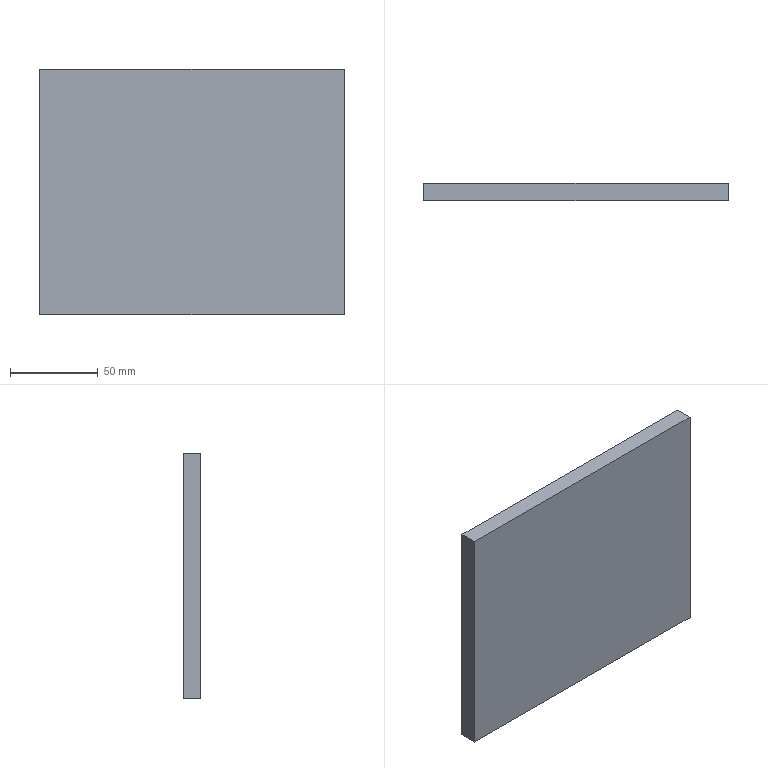Component | SolidWorks | SupportPlate-3 | 1 solid | 6 faces | box 174 x 10 x 140 mm | volume 243600 mm3 | plane 6
build123d program:
from build123d import *

# Parameters (mm, degrees)
SKETCH1_W           = 174
SKETCH1_H           = 140
BOSS_EXTRUDE1_DEPTH = 10


with BuildPart() as part:
    # Sketch1 → Boss-Extrude1 (new body)
    with BuildSketch(Plane.XY):
        with Locations((-218.265, 14.821)):
            Rectangle(SKETCH1_W, SKETCH1_H)
    extrude(amount=BOSS_EXTRUDE1_DEPTH)


solid = part.part

# Placed as in the assembly
solid = solid.moved(Location((218.265, 195, -28.821), (90, 0, 0)))
STEP:
#1=CARTESIAN_POINT('',(3.425,7.283,2.205));
#2=VERTEX_POINT('',#1);
#3=CARTESIAN_POINT('',(3.425,7.283,-3.307));
#4=VERTEX_POINT('',#3);
#5=CARTESIAN_POINT('',(3.425,7.283,2.205));
#6=DIRECTION('',(0.,0.,-1.));
#7=VECTOR('',#6,39.37);
#8=LINE('',#5,#7);
#9=EDGE_CURVE('',#2,#4,#8,.T.);
#10=ORIENTED_EDGE('',*,*,#9,.T.);
#11=CARTESIAN_POINT('',(3.425,7.677,-3.307));
#12=VERTEX_POINT('',#11);
#13=CARTESIAN_POINT('',(3.425,7.677,-3.307));
#14=DIRECTION('',(0.,-1.,0.));
#15=VECTOR('',#14,39.37);
#16=LINE('',#13,#15);
#17=EDGE_CURVE('',#12,#4,#16,.T.);
#18=ORIENTED_EDGE('',*,*,#17,.F.);
#19=CARTESIAN_POINT('',(3.425,7.677,2.205));
#20=VERTEX_POINT('',#19);
#21=CARTESIAN_POINT('',(3.425,7.677,2.205));
#22=DIRECTION('',(0.,0.,-1.));
#23=VECTOR('',#22,39.37);
#24=LINE('',#21,#23);
#25=EDGE_CURVE('',#20,#12,#24,.T.);
#26=ORIENTED_EDGE('',*,*,#25,.F.);
#27=CARTESIAN_POINT('',(3.425,7.677,2.205));
#28=DIRECTION('',(0.,-1.,0.));
#29=VECTOR('',#28,39.37);
#30=LINE('',#27,#29);
#31=EDGE_CURVE('',#20,#2,#30,.T.);
#32=ORIENTED_EDGE('',*,*,#31,.T.);
#33=EDGE_LOOP('',(#10,#18,#26,#32));
#34=FACE_OUTER_BOUND('',#33,.T.);
#35=CARTESIAN_POINT('',(3.425,7.677,2.205));
#36=DIRECTION('',(-1.,0.,0.));
#37=DIRECTION('',(0.,1.,0.));
#38=AXIS2_PLACEMENT_3D('',#35,#36,#37);
#39=PLANE('',#38);
#40=ADVANCED_FACE('',(#34),#39,.F.);
#41=CARTESIAN_POINT('',(-3.425,7.283,-3.307));
#42=VERTEX_POINT('',#41);
#43=CARTESIAN_POINT('',(3.425,7.283,-3.307));
#44=DIRECTION('',(-1.,0.,0.));
#45=VECTOR('',#44,39.37);
#46=LINE('',#43,#45);
#47=EDGE_CURVE('',#4,#42,#46,.T.);
#48=ORIENTED_EDGE('',*,*,#47,.T.);
#49=CARTESIAN_POINT('',(-3.425,7.677,-3.307));
#50=VERTEX_POINT('',#49);
#51=CARTESIAN_POINT('',(-3.425,7.677,-3.307));
#52=DIRECTION('',(0.,-1.,0.));
#53=VECTOR('',#52,39.37);
#54=LINE('',#51,#53);
#55=EDGE_CURVE('',#50,#42,#54,.T.);
#56=ORIENTED_EDGE('',*,*,#55,.F.);
#57=CARTESIAN_POINT('',(3.425,7.677,-3.307));
#58=DIRECTION('',(-1.,0.,0.));
#59=VECTOR('',#58,39.37);
#60=LINE('',#57,#59);
#61=EDGE_CURVE('',#12,#50,#60,.T.);
#62=ORIENTED_EDGE('',*,*,#61,.F.);
#63=ORIENTED_EDGE('',*,*,#17,.T.);
#64=EDGE_LOOP('',(#48,#56,#62,#63));
#65=FACE_OUTER_BOUND('',#64,.T.);
#66=CARTESIAN_POINT('',(3.425,7.677,-3.307));
#67=DIRECTION('',(0.,0.,1.));
#68=DIRECTION('',(0.,-1.,0.));
#69=AXIS2_PLACEMENT_3D('',#66,#67,#68);
#70=PLANE('',#69);
#71=ADVANCED_FACE('',(#65),#70,.F.);
#72=CARTESIAN_POINT('',(-3.425,7.283,2.205));
#73=VERTEX_POINT('',#72);
#74=CARTESIAN_POINT('',(-3.425,7.283,2.205));
#75=DIRECTION('',(0.,0.,1.));
#76=VECTOR('',#75,39.37);
#77=LINE('',#74,#76);
#78=EDGE_CURVE('',#42,#73,#77,.T.);
#79=ORIENTED_EDGE('',*,*,#78,.T.);
#80=CARTESIAN_POINT('',(-3.425,7.677,2.205));
#81=VERTEX_POINT('',#80);
#82=CARTESIAN_POINT('',(-3.425,7.677,2.205));
#83=DIRECTION('',(0.,-1.,0.));
#84=VECTOR('',#83,39.37);
#85=LINE('',#82,#84);
#86=EDGE_CURVE('',#81,#73,#85,.T.);
#87=ORIENTED_EDGE('',*,*,#86,.F.);
#88=CARTESIAN_POINT('',(-3.425,7.677,2.205));
#89=DIRECTION('',(0.,0.,1.));
#90=VECTOR('',#89,39.37);
#91=LINE('',#88,#90);
#92=EDGE_CURVE('',#50,#81,#91,.T.);
#93=ORIENTED_EDGE('',*,*,#92,.F.);
#94=ORIENTED_EDGE('',*,*,#55,.T.);
#95=EDGE_LOOP('',(#79,#87,#93,#94));
#96=FACE_OUTER_BOUND('',#95,.T.);
#97=CARTESIAN_POINT('',(-3.425,7.677,2.205));
#98=DIRECTION('',(1.,0.,0.));
#99=DIRECTION('',(0.,-1.,0.));
#100=AXIS2_PLACEMENT_3D('',#97,#98,#99);
#101=PLANE('',#100);
#102=ADVANCED_FACE('',(#96),#101,.F.);
#103=CARTESIAN_POINT('',(3.425,7.283,2.205));
#104=DIRECTION('',(1.,0.,0.));
#105=VECTOR('',#104,39.37);
#106=LINE('',#103,#105);
#107=EDGE_CURVE('',#73,#2,#106,.T.);
#108=ORIENTED_EDGE('',*,*,#107,.T.);
#109=ORIENTED_EDGE('',*,*,#31,.F.);
#110=CARTESIAN_POINT('',(3.425,7.677,2.205));
#111=DIRECTION('',(1.,0.,0.));
#112=VECTOR('',#111,39.37);
#113=LINE('',#110,#112);
#114=EDGE_CURVE('',#81,#20,#113,.T.);
#115=ORIENTED_EDGE('',*,*,#114,.F.);
#116=ORIENTED_EDGE('',*,*,#86,.T.);
#117=EDGE_LOOP('',(#108,#109,#115,#116));
#118=FACE_OUTER_BOUND('',#117,.T.);
#119=CARTESIAN_POINT('',(3.425,7.677,2.205));
#120=DIRECTION('',(0.,0.,-1.));
#121=DIRECTION('',(0.,1.,0.));
#122=AXIS2_PLACEMENT_3D('',#119,#120,#121);
#123=PLANE('',#122);
#124=ADVANCED_FACE('',(#118),#123,.F.);
#125=ORIENTED_EDGE('',*,*,#25,.T.);
#126=ORIENTED_EDGE('',*,*,#61,.T.);
#127=ORIENTED_EDGE('',*,*,#92,.T.);
#128=ORIENTED_EDGE('',*,*,#114,.T.);
#129=EDGE_LOOP('',(#125,#126,#127,#128));
#130=FACE_OUTER_BOUND('',#129,.T.);
#131=CARTESIAN_POINT('',(8.593,7.677,0.03232));
#132=DIRECTION('',(0.,1.,0.));
#133=DIRECTION('',(1.,0.,0.));
#134=AXIS2_PLACEMENT_3D('',#131,#132,#133);
#135=PLANE('',#134);
#136=ADVANCED_FACE('',(#130),#135,.T.);
#137=ORIENTED_EDGE('',*,*,#9,.F.);
#138=ORIENTED_EDGE('',*,*,#107,.F.);
#139=ORIENTED_EDGE('',*,*,#78,.F.);
#140=ORIENTED_EDGE('',*,*,#47,.F.);
#141=EDGE_LOOP('',(#137,#138,#139,#140));
#142=FACE_OUTER_BOUND('',#141,.T.);
#143=CARTESIAN_POINT('',(8.593,7.283,0.03232));
#144=DIRECTION('',(0.,1.,0.));
#145=DIRECTION('',(1.,0.,0.));
#146=AXIS2_PLACEMENT_3D('',#143,#144,#145);
#147=PLANE('',#146);
#148=ADVANCED_FACE('',(#142),#147,.F.);
#149=CLOSED_SHELL('',(#40,#71,#102,#124,#136,#148));
#150=MANIFOLD_SOLID_BREP('',#149);
#151=CARTESIAN_POINT('',(0.,0.,0.));
#152=DIRECTION('',(0.,0.,1.));
#153=DIRECTION('',(1.,0.,0.));
#154=AXIS2_PLACEMENT_3D('',#151,#152,#153);
#155=(LENGTH_UNIT()NAMED_UNIT(*)SI_UNIT($,.METRE.));
#156=LENGTH_MEASURE_WITH_UNIT(LENGTH_MEASURE(0.0254),#155);
#157=DIMENSIONAL_EXPONENTS(1.,0.,0.,0.,0.,0.,0.);
#158=(CONVERSION_BASED_UNIT('',#156)LENGTH_UNIT()NAMED_UNIT(#157));
#159=UNCERTAINTY_MEASURE_WITH_UNIT(LENGTH_MEASURE(0.00001),#158,'','');
#160=(NAMED_UNIT(*)PLANE_ANGLE_UNIT()SI_UNIT($,.RADIAN.));
#161=(NAMED_UNIT(*)SI_UNIT($,.STERADIAN.)SOLID_ANGLE_UNIT());
#162=(GEOMETRIC_REPRESENTATION_CONTEXT(3)GLOBAL_UNCERTAINTY_ASSIGNED_CONTEXT((#159))GLOBAL_UNIT_ASSIGNED_CONTEXT((#158,#160,#161))REPRESENTATION_CONTEXT('',''));
#163=ADVANCED_BREP_SHAPE_REPRESENTATION('',(#150,#154),#162);
#164=COLOUR_RGB('',0.7922,0.8196,0.9333);
#165=FILL_AREA_STYLE_COLOUR('',#164);
#166=FILL_AREA_STYLE('',(#165));
#167=SURFACE_STYLE_FILL_AREA(#166);
#168=SURFACE_SIDE_STYLE('',(#167));
#169=SURFACE_STYLE_USAGE(.BOTH.,#168);
#170=PRESENTATION_STYLE_ASSIGNMENT((#169));
#171=STYLED_ITEM('',(#170),#150);
#172=(LENGTH_UNIT()NAMED_UNIT(*)SI_UNIT($,.METRE.));
#173=LENGTH_MEASURE_WITH_UNIT(LENGTH_MEASURE(0.0254),#172);
#174=DIMENSIONAL_EXPONENTS(1.,0.,0.,0.,0.,0.,0.);
#175=(CONVERSION_BASED_UNIT('',#173)LENGTH_UNIT()NAMED_UNIT(#174));
#176=UNCERTAINTY_MEASURE_WITH_UNIT(LENGTH_MEASURE(0.00001),#175,'','');
#177=(NAMED_UNIT(*)PLANE_ANGLE_UNIT()SI_UNIT($,.RADIAN.));
#178=(NAMED_UNIT(*)SI_UNIT($,.STERADIAN.)SOLID_ANGLE_UNIT());
#179=(GEOMETRIC_REPRESENTATION_CONTEXT(3)GLOBAL_UNCERTAINTY_ASSIGNED_CONTEXT((#176))GLOBAL_UNIT_ASSIGNED_CONTEXT((#175,#177,#178))REPRESENTATION_CONTEXT('',''));
#180=MECHANICAL_DESIGN_GEOMETRIC_PRESENTATION_REPRESENTATION('',(#171),#179);
#181=PRESENTATION_LAYER_ASSIGNMENT('','',(#171));